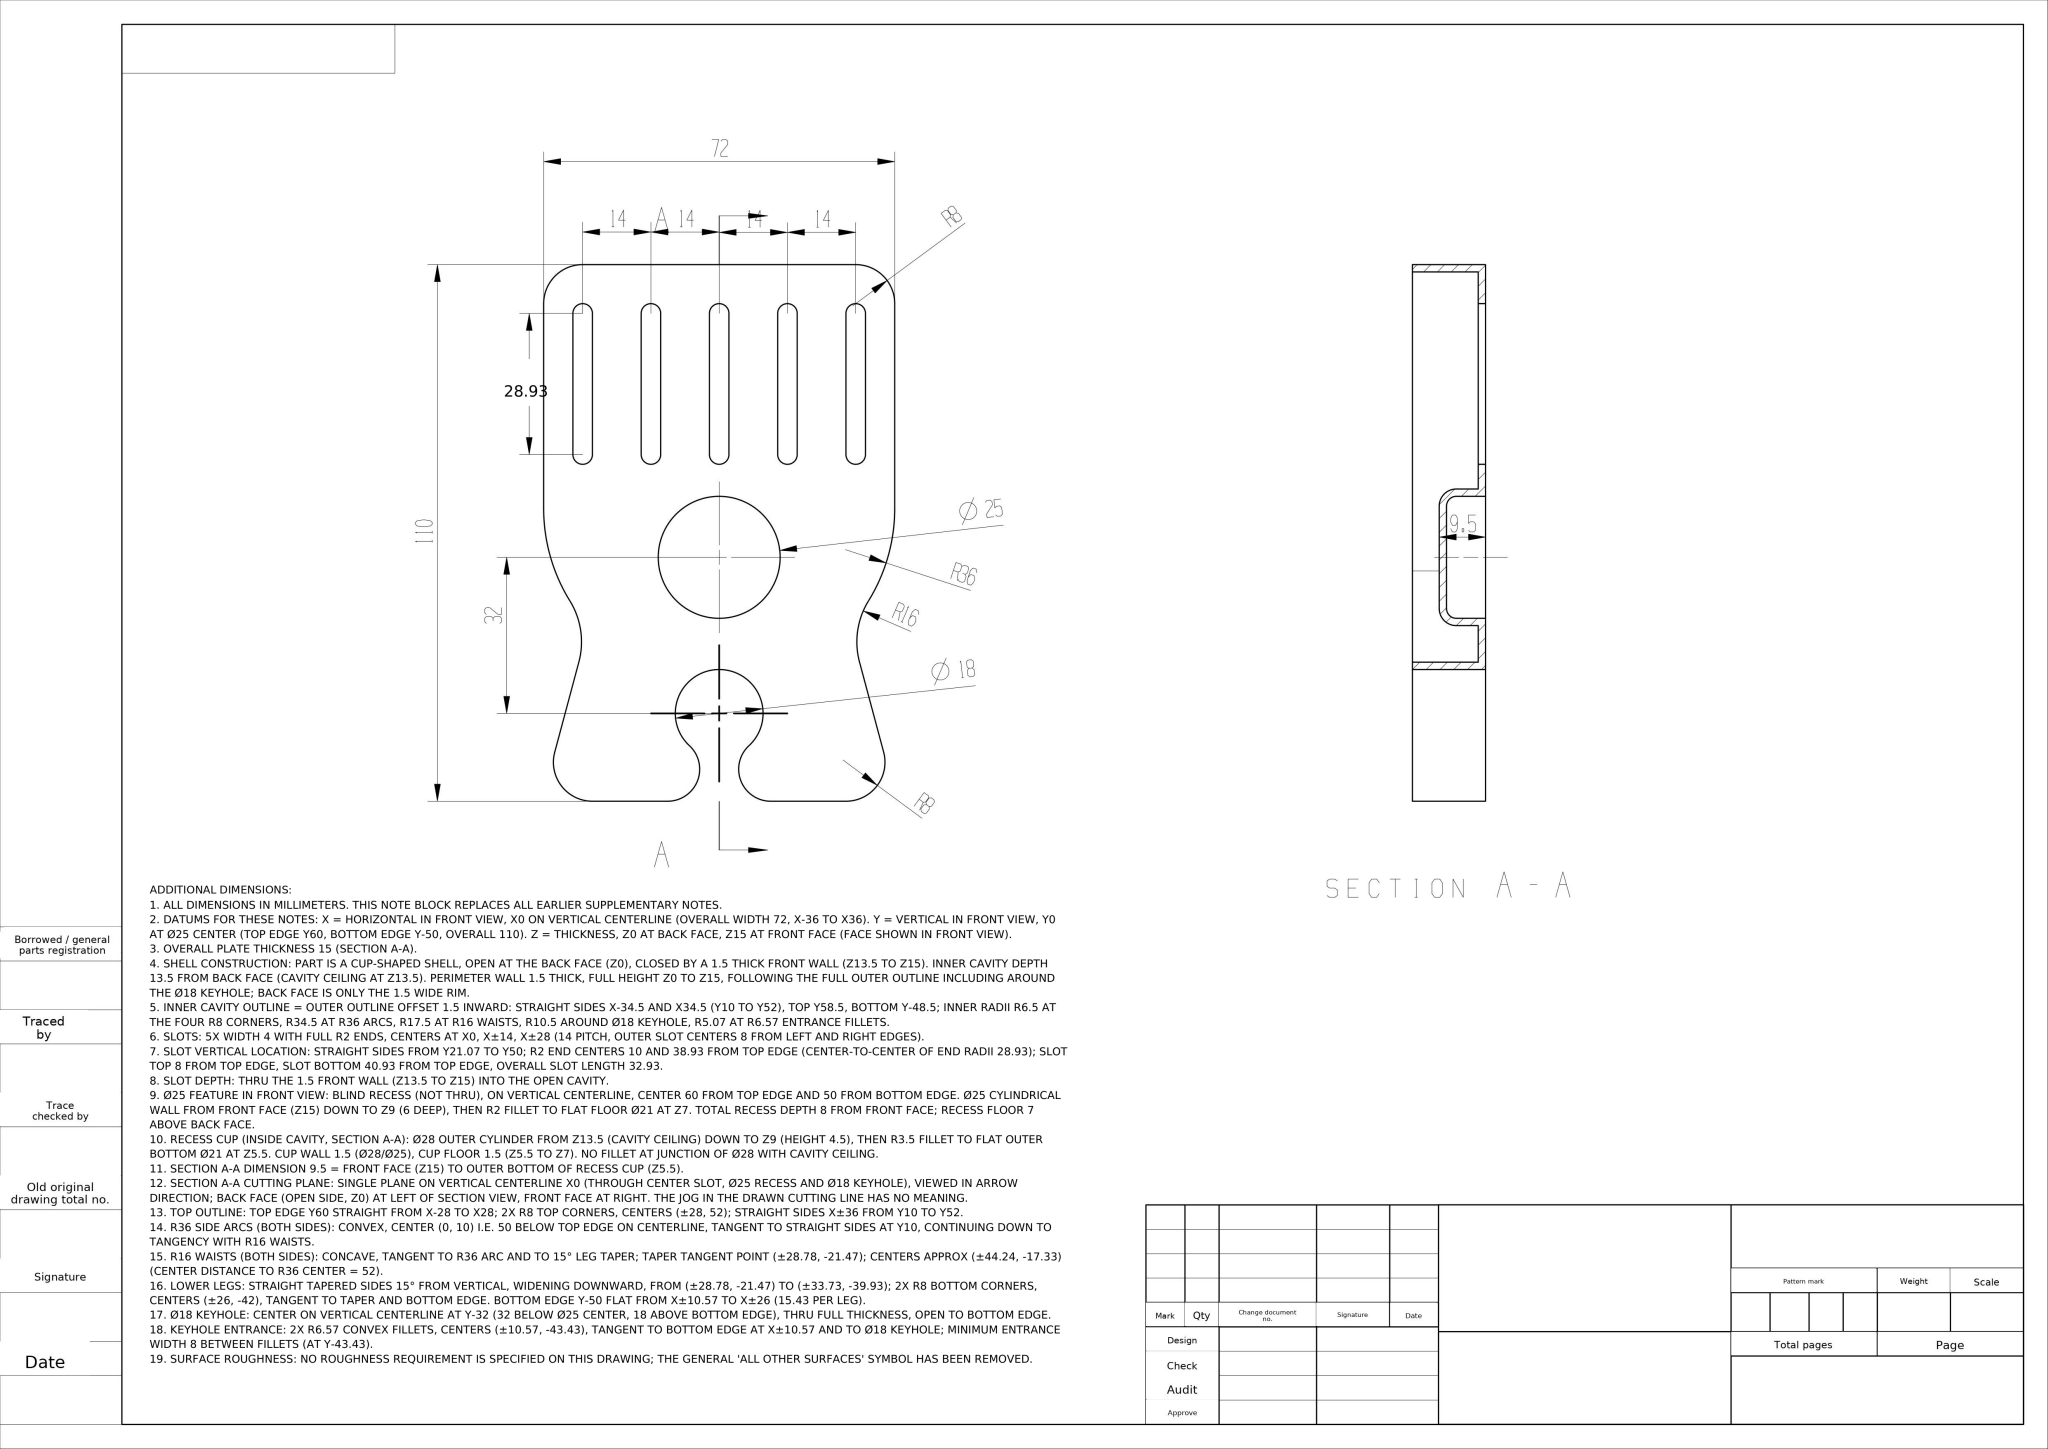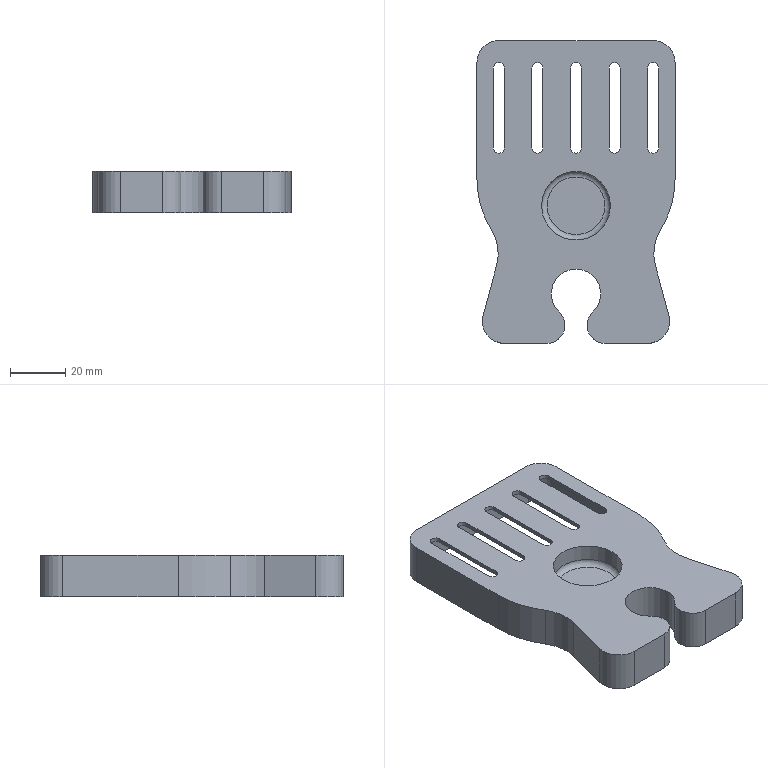Part | NX | mm | 1 solid | 65 faces | box 72 x 110 x 15 mm | volume 18549 mm3 | cylinder 34 | plane 29 | torus 2 | commonest cylinder face diameters 4 x10 16 x4 13 x4 72 x2 32 x2 13.137 x2 69 x2 35 x2